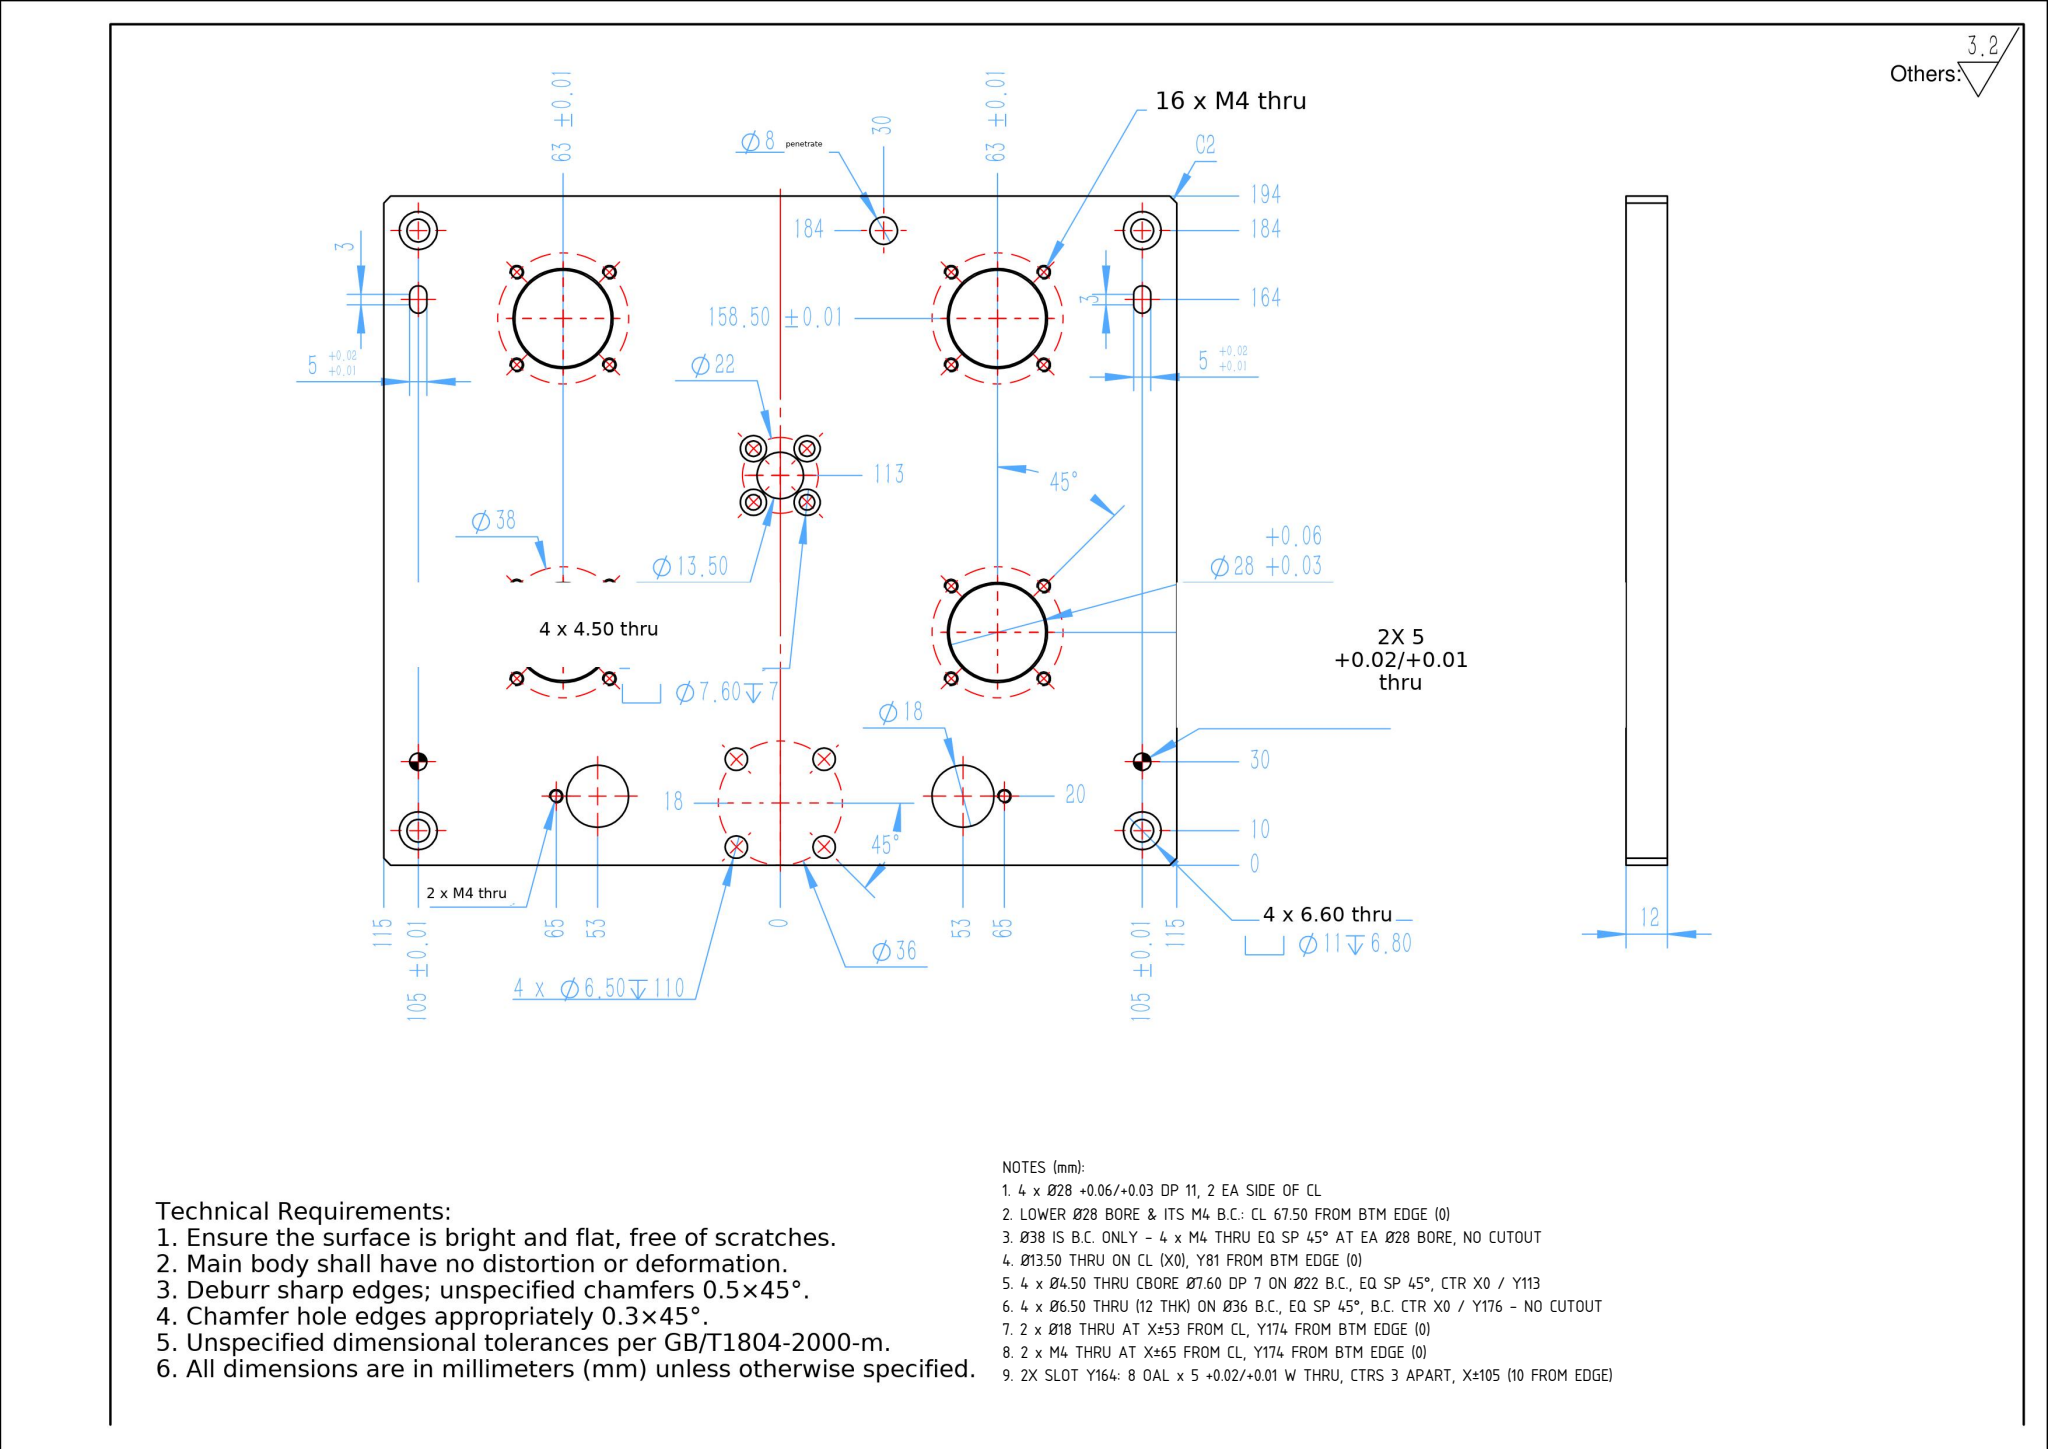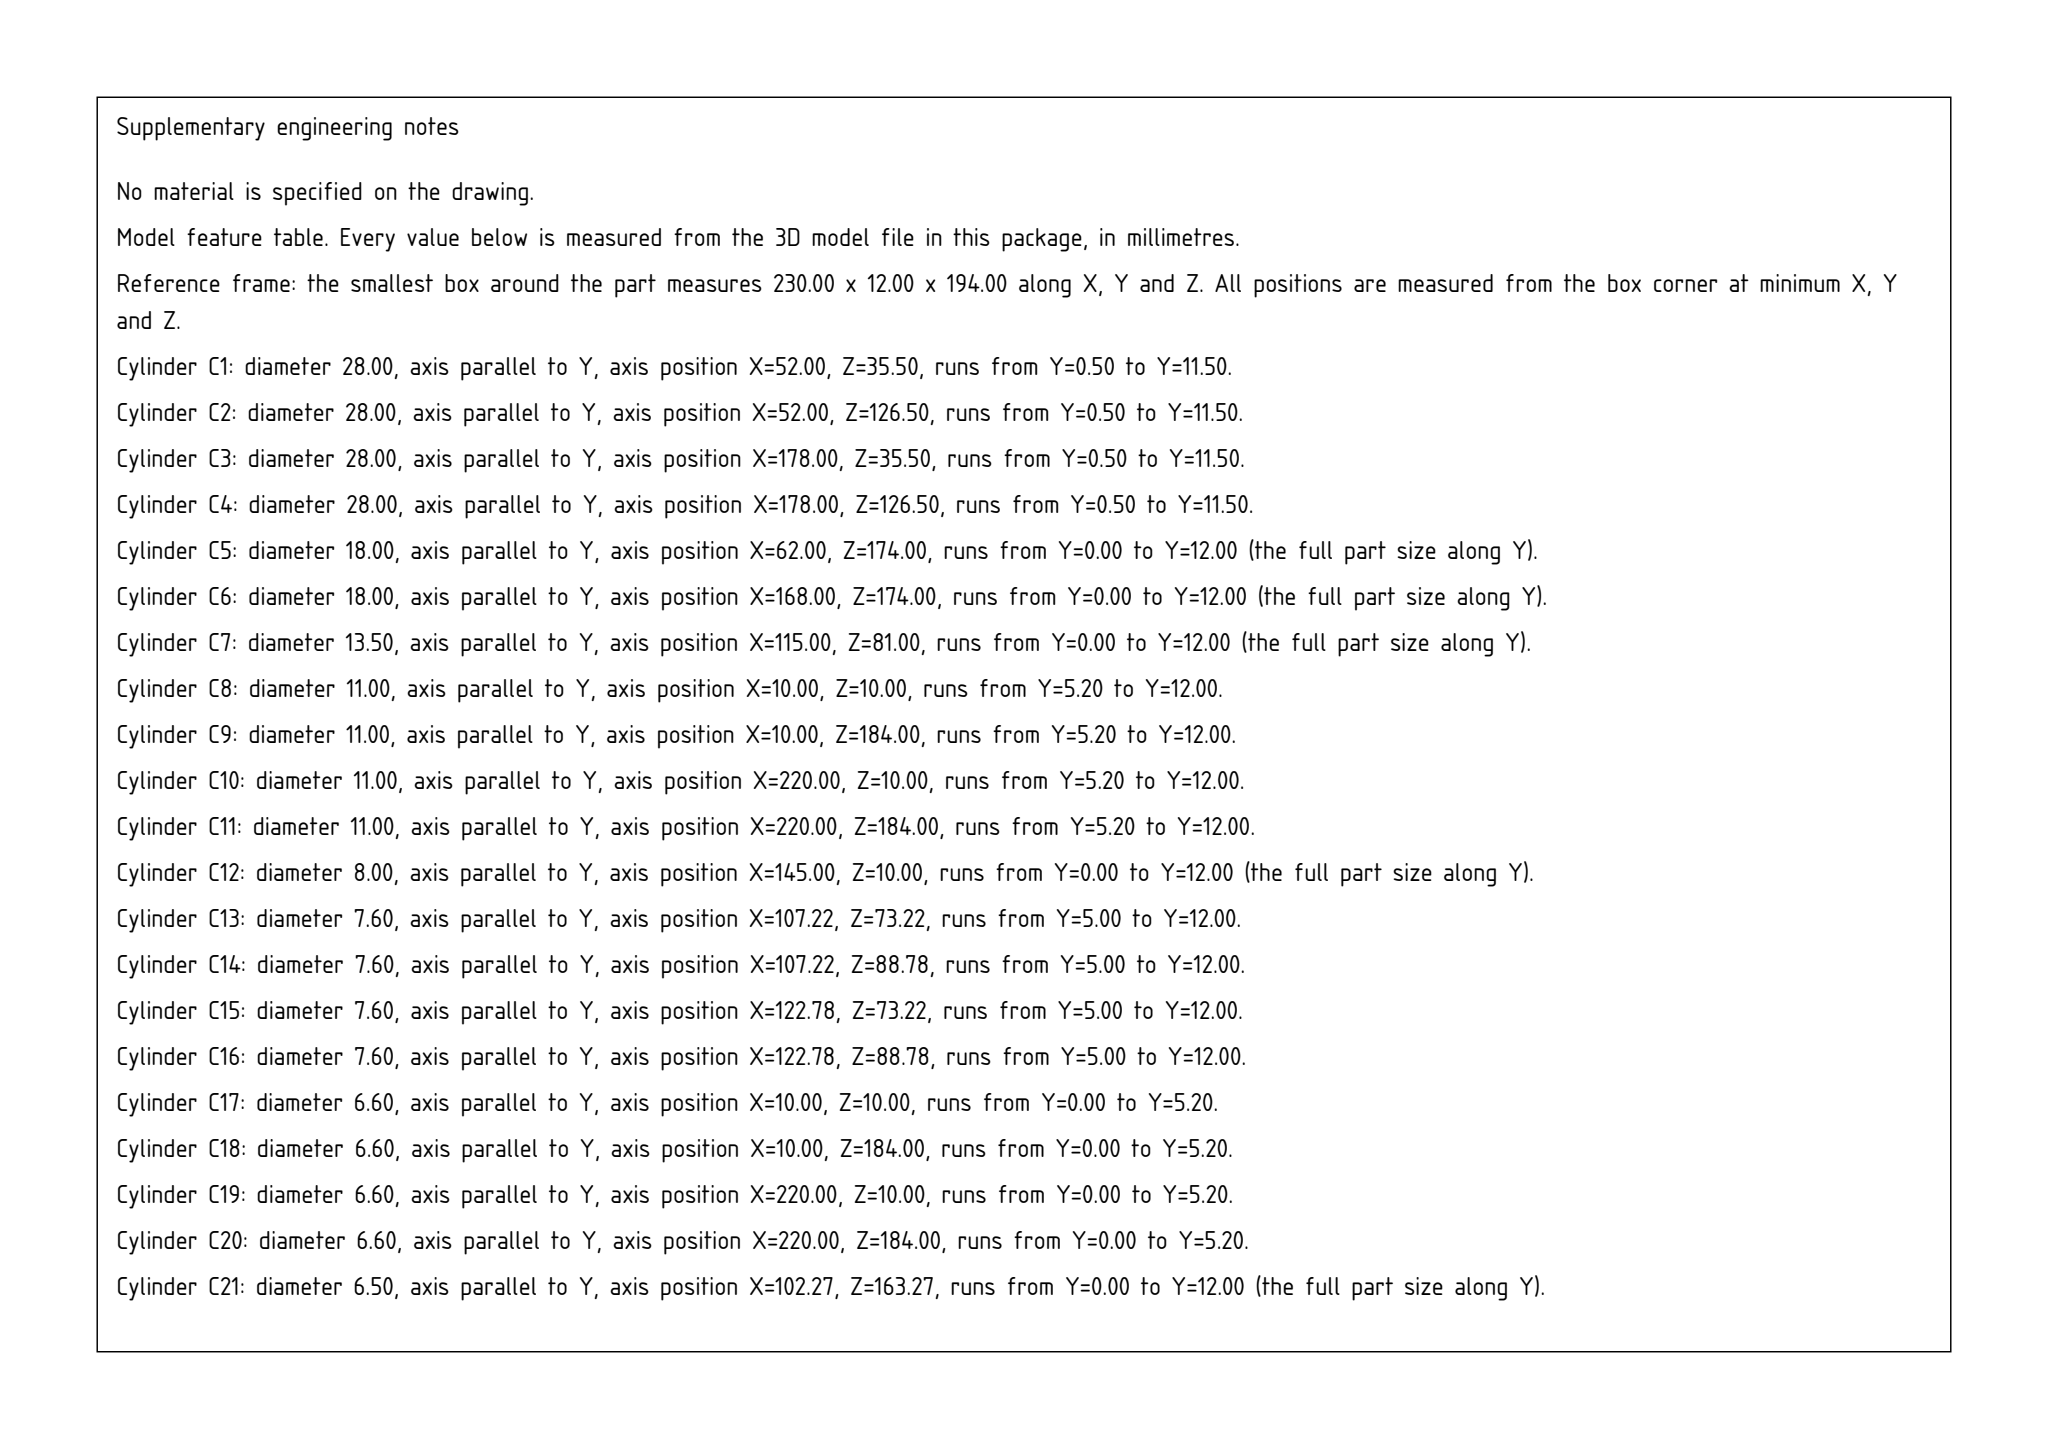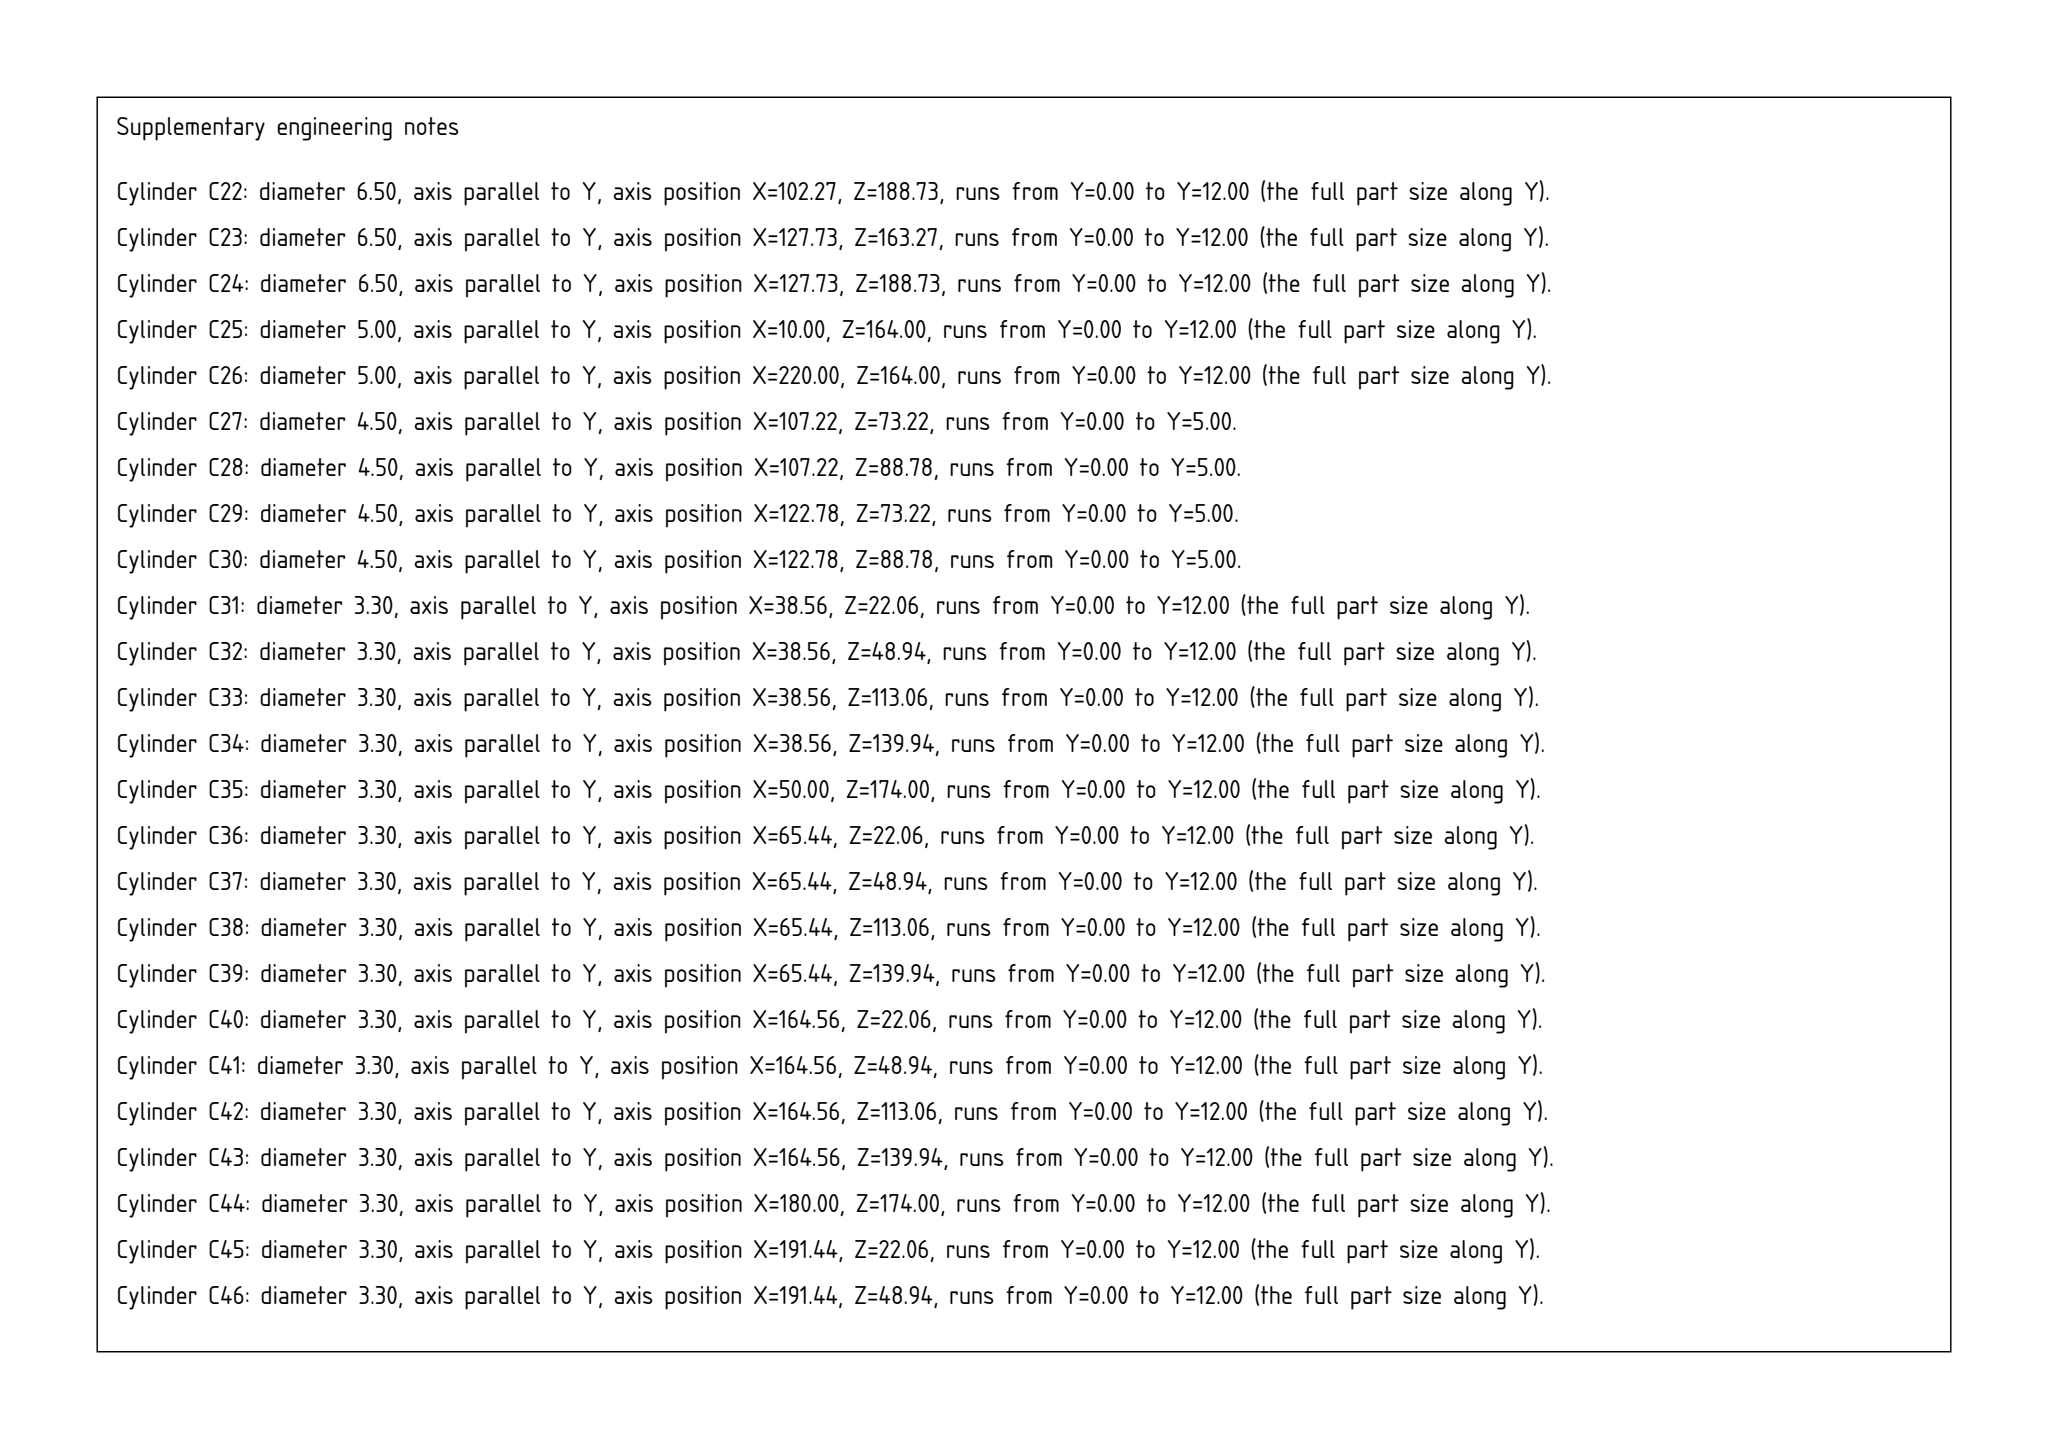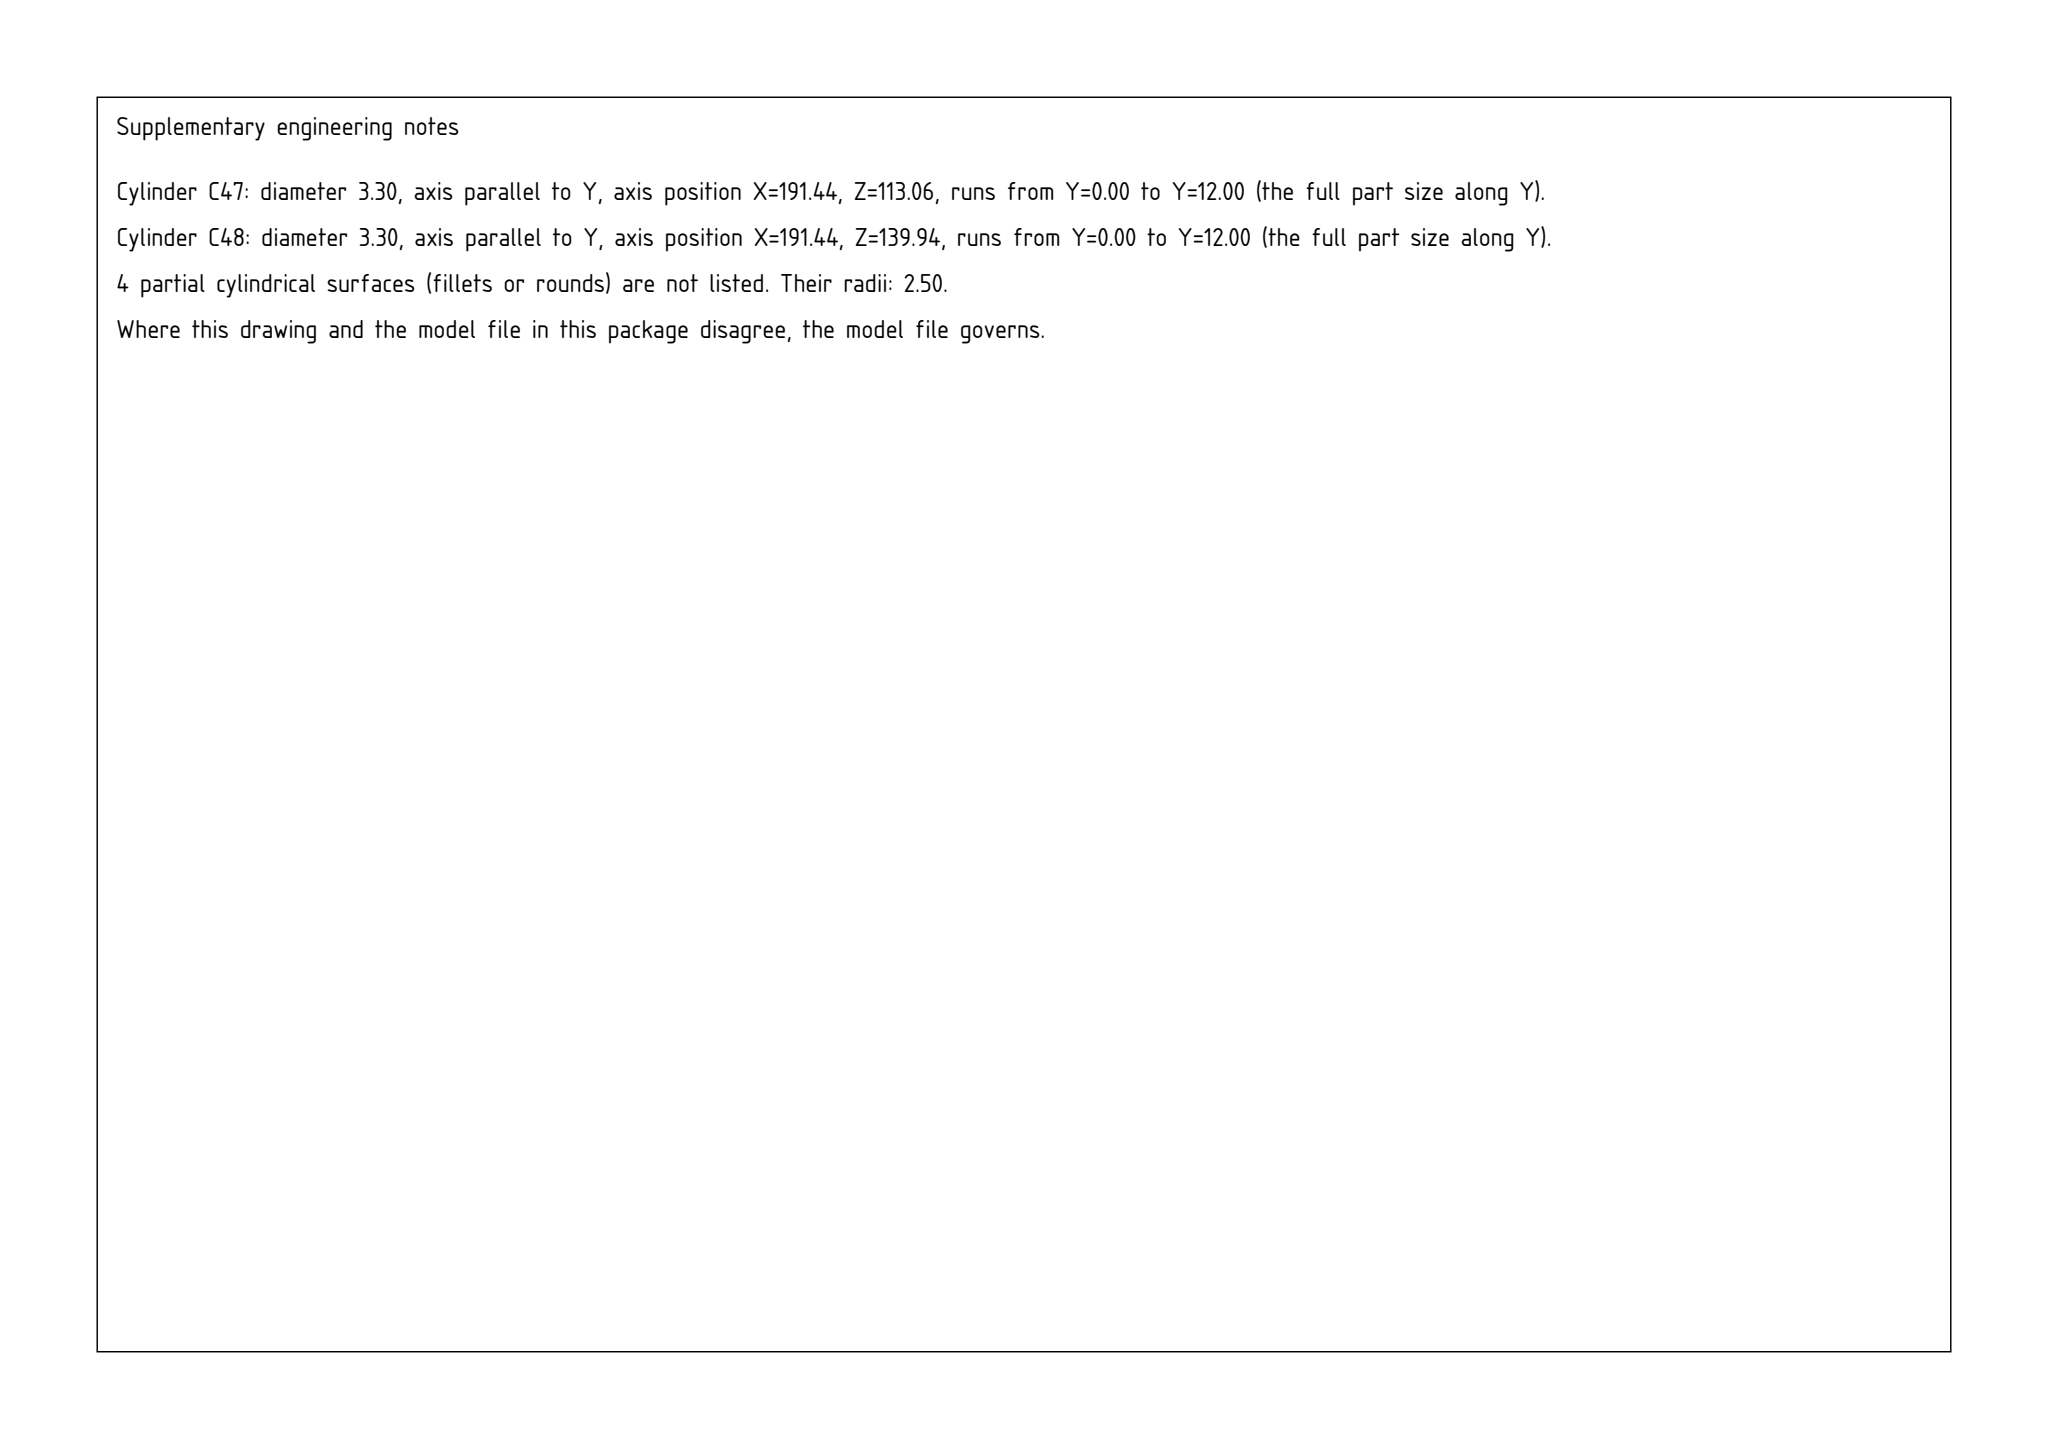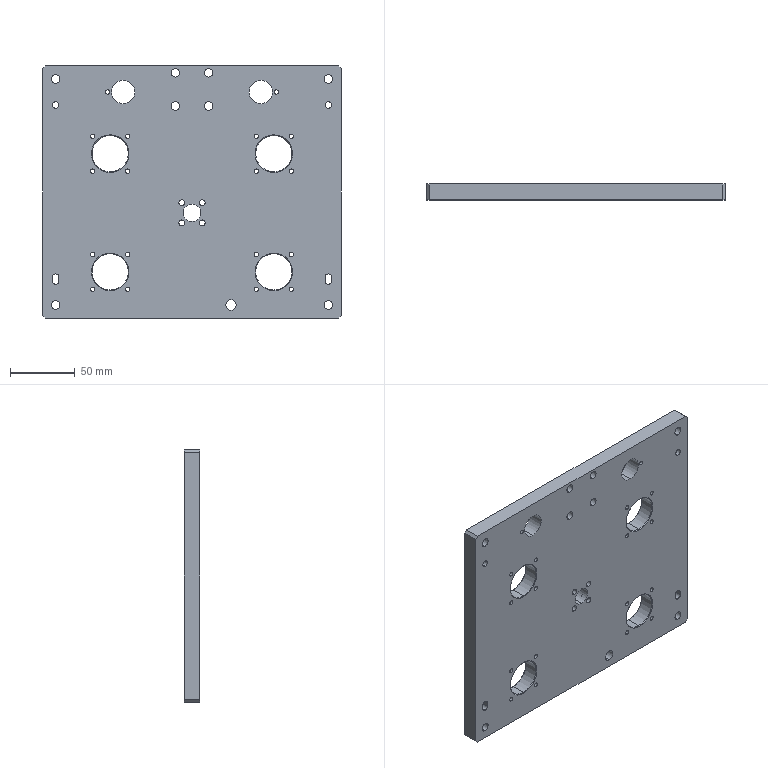Part | SolidWorks | mm | 1 solid | 140 faces | box 230 x 12 x 194 mm | volume 487643 mm3 | cylinder 102 | plane 22 | cone 16 | commonest cylinder face diameters 3.3 x36 5 x10 6.5 x8 11 x8 6.6 x8 7.6 x8 4.5 x8 28 x8
Drawing notes:
4 x Ø28 +0.06/+0.03 DP 11, 2 EA SIDE OF CL | from the solid: Ø28 cyl len 11 at (52,35.5)(52,126.5)(178,35.5)(178,126.5)
LOWER Ø28 BORE & ITS M4 B.C.: CL 67.50 FROM BTM EDGE (0) | from the solid: Ø28 cyl at z=126.5 -> 194-126.5 = 67.50 from datum edge
Ø38 IS B.C. ONLY - 4 x M4 THRU EQ SP 45° AT EA Ø28 BORE, NO CUTOUT | from the solid: Ø3.3 holes at ±13.44 x/z about each bore ctr -> R19, Ø38 B.C.; no Ø38 face
Ø13.50 THRU ON CL (X0), Y81 FROM BTM EDGE (0) | from the solid: cyl Ø13.5 axis y at (115,81), len 12 = plate thk
4 x Ø4.50 THRU CBORE Ø7.60 DP 7 ON Ø22 B.C., EQ SP 45°, CTR X0 / Y113 | from the solid: Ø4.5 thru + Ø7.6 len 7 at (107.22/122.78, 73.22/88.78), ctr (115,81), R11
4 x Ø6.50 THRU (12 THK) ON Ø36 B.C., EQ SP 45°, B.C. CTR X0 / Y176 - NO CUTOUT | from the solid: Ø6.5 cyls len 12 at (102.27/127.73, 163.27/188.73), ctr (115,176); no Ø36 face
2 x Ø18 THRU AT X±53 FROM CL, Y174 FROM BTM EDGE (0) | from the solid: Ø18 cyls len 12 at (62,174) & (168,174), CL x=115
2 x M4 THRU AT X±65 FROM CL, Y174 FROM BTM EDGE (0) | from the solid: Ø3.3 thru cyls at (50,174) & (180,174), CL x=115
2X SLOT Y164: 8 OAL x 5 +0.02/+0.01 W THRU, CTRS 3 APART, X±105 (10 FROM EDGE) | from the solid: Ø5 thru pairs z=28.5/31.5 at x=10 & 220, flats x=7.5/12.5; bbox X 0-230
build123d program:
from build123d import *

# Parameters (mm, degrees)
SKETCH1_W                                         = 230
SKETCH1_H                                         = 194
BOSS_EXTRUDE1_DEPTH                               = 12
SKETCH2_R                                         = 14
CUT_EXTRUDE1_DEPTH                                = 151.924
M4_TAPPED_HOLE1_D                                 = 3.3
SKETCH5_R                                         = 6.75
CUT_EXTRUDE2_DEPTH                                = 151.924
HOLE_SIZE_ACCORDING_TO_TYPE_0_OF_HEXA_D           = 4.5
HOLE_SIZE_ACCORDING_TO_TYPE_0_OF_HEXA_CBORE_D     = 7.6
HOLE_SIZE_ACCORDING_TO_TYPE_0_OF_HEXA_CBORE_DEPTH = 7
CHAMFER1_SIZE                                     = 2
HOLE_SIZE_ACCORDING_TO_TYPE_2_OF_HEXA_D           = 6.6
HOLE_SIZE_ACCORDING_TO_TYPE_2_OF_HEXA_CBORE_D     = 11
HOLE_SIZE_ACCORDING_TO_TYPE_2_OF_HEXA_CBORE_DEPTH = 6.8
F_6_5_6_5_DIAMETER_HOLE1_D                        = 6.5
F_6_5_6_5_DIAMETER_HOLE1_DEPTH                    = 110
F_6_5_6_5_DIAMETER_HOLE1_TIP                      = 1.953
SKETCH13_R                                        = 4
CUT_EXTRUDE4_DEPTH                                = 151.924
SKETCH14_R                                        = 9
CUT_EXTRUDE5_DEPTH                                = 151.924
M4_TAPPED_HOLE2_D                                 = 3.3
CHAMFER2_SIZE                                     = 0.5
SKETCH19_R                                        = 2.5
CUT_EXTRUDE6_DEPTH                                = 151.924


with BuildPart() as part:
    # Sketch1 → Boss-Extrude1 (new body)
    with BuildSketch(Plane(origin=(0, 0, 0), x_dir=(1, 0, 0), z_dir=(0, 1, 0))):
        Rectangle(SKETCH1_W, SKETCH1_H)
    extrude(amount=BOSS_EXTRUDE1_DEPTH)

    # Sketch2 → Cut-Extrude1 (cut, through all)
    with BuildSketch(Plane(origin=(0, 12, 0), x_dir=(1, 0, 0), z_dir=(0, 1, 0))):
        with Locations(Location((-63, 61.5, 0), (0, 0, 270))):
            Circle(SKETCH2_R)
        with Locations(Location((63, 61.5, 0), (0, 0, 90))):
            Circle(SKETCH2_R)
        with Locations(Location((-63, -29.5, 0), (0, 0, 270))):
            Circle(SKETCH2_R)
        with Locations(Location((63, -29.5, 0), (0, 0, 270))):
            Circle(SKETCH2_R)
    extrude(amount=-CUT_EXTRUDE1_DEPTH, mode=Mode.SUBTRACT)

    # M4 Tapped Hole1 (through all)
    with Locations(Plane(origin=(0, 12, 0), x_dir=(1, 0, 0), z_dir=(0, 1, 0))):
        with Locations((76.435, 74.935), (49.565, 74.935), (49.565, 48.065), (76.435, 48.065), (-49.565, 74.935), (-76.435, 74.935), (-76.435, 48.065), (-49.565, 48.065), (-49.565, -16.065), (-76.435, -16.065), (-76.435, -42.935), (-49.565, -42.935), (49.565, -16.065), (49.565, -42.935), (76.435, -42.935), (76.435, -16.065)):
            Hole(M4_TAPPED_HOLE1_D / 2)

    # Sketch5 → Cut-Extrude2 (cut, through all)
    with BuildSketch(Plane(origin=(0, 12, 0), x_dir=(1, 0, 0), z_dir=(0, 1, 0))):
        with Locations(Location((0, 16, 0), (0, 0, 270))):
            Circle(SKETCH5_R)
    extrude(amount=-CUT_EXTRUDE2_DEPTH, mode=Mode.SUBTRACT)

    # Hole Size _ according to_ Type 0 of Hexa (through all)
    with Locations(Plane(origin=(0, 12, 0), x_dir=(1, 0, 0), z_dir=(0, 1, 0))):
        with Locations((-7.778, 23.778), (-7.778, 8.222), (7.778, 8.222), (7.778, 23.778)):
            CounterBoreHole(HOLE_SIZE_ACCORDING_TO_TYPE_0_OF_HEXA_D / 2, HOLE_SIZE_ACCORDING_TO_TYPE_0_OF_HEXA_CBORE_D / 2, HOLE_SIZE_ACCORDING_TO_TYPE_0_OF_HEXA_CBORE_DEPTH)

    # Chamfer1
    chamfer1_edges = [part.edges().sort_by_distance(p)[0] for p in [
        (115, 6, 97),
        (-115, 6, 97),
        (-115, 6, -97),
        (115, 6, -97),
    ]]
    chamfer(chamfer1_edges, length=CHAMFER1_SIZE)

    # Hole Size _ according to_ Type 2 of Hexa (through all)
    with Locations(Plane(origin=(0, 12, 0), x_dir=(-1, 0, 0), z_dir=(0, 1, 0))):
        with Locations((105, 87), (105, -87), (-105, -87), (-105, 87)):
            CounterBoreHole(HOLE_SIZE_ACCORDING_TO_TYPE_2_OF_HEXA_D / 2, HOLE_SIZE_ACCORDING_TO_TYPE_2_OF_HEXA_CBORE_D / 2, HOLE_SIZE_ACCORDING_TO_TYPE_2_OF_HEXA_CBORE_DEPTH)

    # 6.5 _6.5_ Diameter Hole1
    with Locations(Plane(origin=(0, 0, 0), x_dir=(-1, 0, 0), z_dir=(0, -1, 0))):
        with Locations((-12.728, -91.728), (12.728, -66.272), (12.728, -91.728), (-12.728, -66.272)):
            Hole(F_6_5_6_5_DIAMETER_HOLE1_D / 2, depth=F_6_5_6_5_DIAMETER_HOLE1_DEPTH)
            with Locations((0, 0, -(F_6_5_6_5_DIAMETER_HOLE1_DEPTH + F_6_5_6_5_DIAMETER_HOLE1_TIP / 2))):  # 118° drill point
                Cone(0, F_6_5_6_5_DIAMETER_HOLE1_D / 2, F_6_5_6_5_DIAMETER_HOLE1_TIP, mode=Mode.SUBTRACT)

    # Sketch13 → Cut-Extrude4 (cut, through all)
    with BuildSketch(Plane(origin=(0, 12, 0), x_dir=(1, 0, 0), z_dir=(0, 1, 0))):
        with Locations(Location((30, 87, 0), (0, 0, 270))):
            Circle(SKETCH13_R)
    extrude(amount=-CUT_EXTRUDE4_DEPTH, mode=Mode.SUBTRACT)

    # Sketch14 → Cut-Extrude5 (cut, through all)
    with BuildSketch(Plane(origin=(0, 12, 0), x_dir=(1, 0, 0), z_dir=(0, 1, 0))):
        with Locations(Location((-53, -77, 0), (0, 0, 270))):
            Circle(SKETCH14_R)
        with Locations(Location((53, -77, 0), (0, 0, 270))):
            Circle(SKETCH14_R)
    extrude(amount=-CUT_EXTRUDE5_DEPTH, mode=Mode.SUBTRACT)

    # M4 Tapped Hole2 (through all)
    with Locations(Plane(origin=(0, 12, 0), x_dir=(1, 0, 0), z_dir=(0, 1, 0))):
        with Locations((65, -77), (-65, -77)):
            Hole(M4_TAPPED_HOLE2_D / 2)

    # Chamfer2
    chamfer2_edges = [part.edges().sort_by_distance(p)[0] for p in [
        (-63, 0, -75.5),
        (-63, 12, -75.5),
        (63, 0, -47.5),
        (63, 12, -47.5),
        (-63, 0, 15.5),
        (-63, 12, 15.5),
        (63, 0, 15.5),
        (63, 12, 15.5),
    ]]
    chamfer(chamfer2_edges, length=CHAMFER2_SIZE)

    # Sketch19 → Cut-Extrude6 (cut, through all)
    with BuildSketch(Plane.XZ):
        with Locations(Location((-105, 67, 0), (0, 0, 270))):
            Circle(SKETCH19_R)
        with Locations(Location((105, 67, 0), (0, 0, 270))):
            Circle(SKETCH19_R)
        with BuildLine():
            Line((102.5, -68.5), (102.5, -65.5))
            ThreePointArc((102.5, -65.5), (105, -63), (107.5, -65.5))
            Line((107.5, -65.5), (107.5, -68.5))
            ThreePointArc((107.5, -68.5), (105, -71), (102.5, -68.5))
        make_face()
        with BuildLine():
            Line((-102.5, -65.5), (-102.5, -68.5))
            ThreePointArc((-102.5, -68.5), (-105, -71), (-107.5, -68.5))
            Line((-107.5, -68.5), (-107.5, -65.5))
            ThreePointArc((-107.5, -65.5), (-105, -63), (-102.5, -65.5))
        make_face()
    extrude(amount=-CUT_EXTRUDE6_DEPTH, mode=Mode.SUBTRACT)


solid = part.part